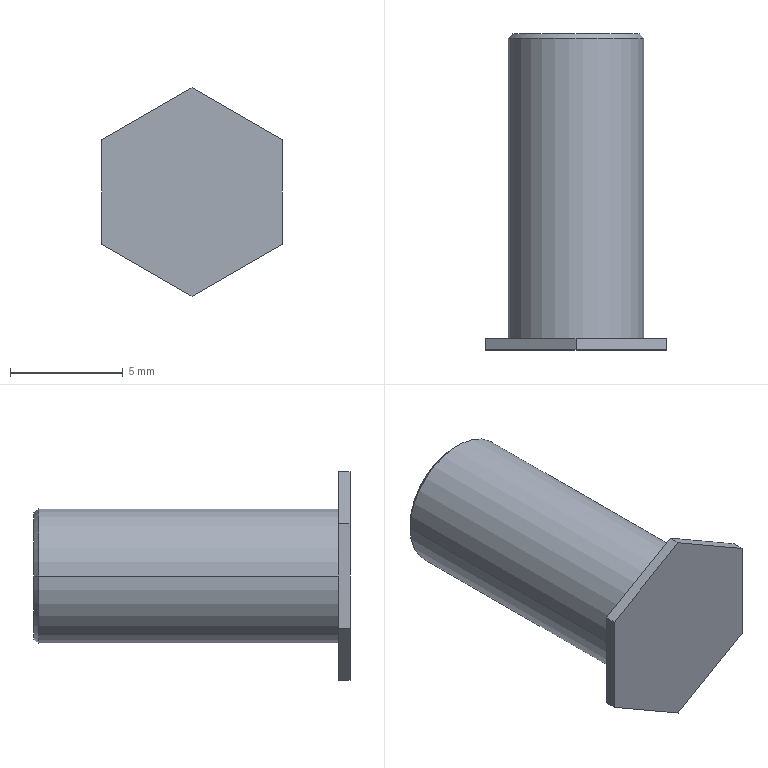Component | SolidWorks | FrontDoorAssembly-1_FrontDoorWelding-1_FrontDoorFrame(Riveted)PG50-02-101-1_FH-M6-14-1 | 1 solid | 13 faces | box 8 x 14 x 9.24 mm | volume 409 mm3 | plane 9 | cone 2 | cylinder 2 | commonest cylinder face diameters 6 x2
build123d program:
from build123d import *

# Parameters (mm, degrees)
BOSS_EXTRUDE1_DEPTH = 0.5
SKETCH2_R           = 3
BOSS_EXTRUDE2_DEPTH = 13.5
CHAMFER1_SIZE       = 0.2


with BuildPart() as part:
    # Sketch1 → Boss-Extrude1 (new body)
    with BuildSketch(Plane.XY):
        Polygon((0, 4.619), (-4, 2.309), (-4, -2.309), (0, -4.619), (4, -2.309), (4, 2.309), align=None)
    extrude(amount=BOSS_EXTRUDE1_DEPTH)

    # Sketch2 → Boss-Extrude2 (add)
    with BuildSketch(Plane.XY.offset(0.5)):
        Circle(SKETCH2_R)
    extrude(amount=BOSS_EXTRUDE2_DEPTH)

    # Chamfer1
    chamfer1_edges = [part.edges().sort_by_distance(p)[0] for p in [
        (-3, 0, 14),
    ]]
    chamfer(chamfer1_edges, length=CHAMFER1_SIZE)


solid = part.part

# Placed as in the assembly
solid = solid.moved(Location((897.314, -283.799, -334.996), (-90, 0, 0)))
STEP:
#1=CARTESIAN_POINT('',(35.438,-10.622,-13.189));
#2=VERTEX_POINT('',#1);
#3=CARTESIAN_POINT('',(35.217,-10.622,-13.189));
#4=VERTEX_POINT('',#3);
#5=CARTESIAN_POINT('',(35.327,-10.622,-13.189));
#6=DIRECTION('',(-0.,1.,0.));
#7=DIRECTION('',(1.,0.,0.));
#8=AXIS2_PLACEMENT_3D('',#5,#6,#7);
#9=CIRCLE('',#8,0.1102);
#10=EDGE_CURVE('',#2,#4,#9,.T.);
#11=ORIENTED_EDGE('',*,*,#10,.F.);
#12=CARTESIAN_POINT('',(35.445,-10.63,-13.189));
#13=VERTEX_POINT('',#12);
#14=CARTESIAN_POINT('',(35.438,-10.622,-13.189));
#15=DIRECTION('',(0.7071,-0.7071,-0.));
#16=VECTOR('',#15,39.37);
#17=LINE('',#14,#16);
#18=EDGE_CURVE('',#2,#13,#17,.T.);
#19=ORIENTED_EDGE('',*,*,#18,.T.);
#20=CARTESIAN_POINT('',(35.209,-10.63,-13.189));
#21=VERTEX_POINT('',#20);
#22=CARTESIAN_POINT('',(35.327,-10.63,-13.189));
#23=DIRECTION('',(0.,-1.,-0.));
#24=DIRECTION('',(1.,0.,0.));
#25=AXIS2_PLACEMENT_3D('',#22,#23,#24);
#26=CIRCLE('',#25,0.1181);
#27=EDGE_CURVE('',#21,#13,#26,.T.);
#28=ORIENTED_EDGE('',*,*,#27,.F.);
#29=CARTESIAN_POINT('',(35.217,-10.622,-13.189));
#30=DIRECTION('',(-0.7071,-0.7071,0.));
#31=VECTOR('',#30,39.37);
#32=LINE('',#29,#31);
#33=EDGE_CURVE('',#4,#21,#32,.T.);
#34=ORIENTED_EDGE('',*,*,#33,.F.);
#35=EDGE_LOOP('',(#11,#19,#28,#34));
#36=FACE_OUTER_BOUND('',#35,.T.);
#37=CARTESIAN_POINT('',(35.327,-10.622,-13.189));
#38=DIRECTION('',(0.,-1.,-0.));
#39=DIRECTION('',(-1.,0.,0.));
#40=AXIS2_PLACEMENT_3D('',#37,#38,#39);
#41=CONICAL_SURFACE('',#40,0.1102,0.7854);
#42=ADVANCED_FACE('',(#36),#41,.T.);
#43=ORIENTED_EDGE('',*,*,#27,.T.);
#44=CARTESIAN_POINT('',(35.445,-11.153,-13.189));
#45=VERTEX_POINT('',#44);
#46=CARTESIAN_POINT('',(35.445,-10.622,-13.189));
#47=DIRECTION('',(0.,-1.,-0.));
#48=VECTOR('',#47,39.37);
#49=LINE('',#46,#48);
#50=EDGE_CURVE('',#13,#45,#49,.T.);
#51=ORIENTED_EDGE('',*,*,#50,.T.);
#52=CARTESIAN_POINT('',(35.209,-11.153,-13.189));
#53=VERTEX_POINT('',#52);
#54=CARTESIAN_POINT('',(35.327,-11.153,-13.189));
#55=DIRECTION('',(-0.,1.,0.));
#56=DIRECTION('',(1.,0.,0.));
#57=AXIS2_PLACEMENT_3D('',#54,#55,#56);
#58=CIRCLE('',#57,0.1181);
#59=EDGE_CURVE('',#45,#53,#58,.T.);
#60=ORIENTED_EDGE('',*,*,#59,.T.);
#61=CARTESIAN_POINT('',(35.209,-10.622,-13.189));
#62=DIRECTION('',(0.,-1.,-0.));
#63=VECTOR('',#62,39.37);
#64=LINE('',#61,#63);
#65=EDGE_CURVE('',#21,#53,#64,.T.);
#66=ORIENTED_EDGE('',*,*,#65,.F.);
#67=EDGE_LOOP('',(#43,#51,#60,#66));
#68=FACE_OUTER_BOUND('',#67,.T.);
#69=CARTESIAN_POINT('',(35.327,-10.622,-13.189));
#70=DIRECTION('',(0.,-1.,-0.));
#71=DIRECTION('',(-1.,0.,0.));
#72=AXIS2_PLACEMENT_3D('',#69,#70,#71);
#73=CYLINDRICAL_SURFACE('',#72,0.1181);
#74=ADVANCED_FACE('',(#68),#73,.T.);
#75=CARTESIAN_POINT('',(35.485,-11.153,-13.28));
#76=VERTEX_POINT('',#75);
#77=CARTESIAN_POINT('',(35.327,-11.153,-13.371));
#78=VERTEX_POINT('',#77);
#79=CARTESIAN_POINT('',(35.485,-11.153,-13.28));
#80=DIRECTION('',(-0.866,-0.,-0.5));
#81=VECTOR('',#80,39.37);
#82=LINE('',#79,#81);
#83=EDGE_CURVE('',#76,#78,#82,.T.);
#84=ORIENTED_EDGE('',*,*,#83,.T.);
#85=CARTESIAN_POINT('',(35.17,-11.153,-13.28));
#86=VERTEX_POINT('',#85);
#87=CARTESIAN_POINT('',(35.327,-11.153,-13.371));
#88=DIRECTION('',(-0.866,-0.,0.5));
#89=VECTOR('',#88,39.37);
#90=LINE('',#87,#89);
#91=EDGE_CURVE('',#78,#86,#90,.T.);
#92=ORIENTED_EDGE('',*,*,#91,.T.);
#93=CARTESIAN_POINT('',(35.17,-11.153,-13.098));
#94=VERTEX_POINT('',#93);
#95=CARTESIAN_POINT('',(35.17,-11.153,-13.28));
#96=DIRECTION('',(-0.,-0.,1.));
#97=VECTOR('',#96,39.37);
#98=LINE('',#95,#97);
#99=EDGE_CURVE('',#86,#94,#98,.T.);
#100=ORIENTED_EDGE('',*,*,#99,.T.);
#101=CARTESIAN_POINT('',(35.327,-11.153,-13.007));
#102=VERTEX_POINT('',#101);
#103=CARTESIAN_POINT('',(35.17,-11.153,-13.098));
#104=DIRECTION('',(0.866,0.,0.5));
#105=VECTOR('',#104,39.37);
#106=LINE('',#103,#105);
#107=EDGE_CURVE('',#94,#102,#106,.T.);
#108=ORIENTED_EDGE('',*,*,#107,.T.);
#109=CARTESIAN_POINT('',(35.485,-11.153,-13.098));
#110=VERTEX_POINT('',#109);
#111=CARTESIAN_POINT('',(35.327,-11.153,-13.007));
#112=DIRECTION('',(0.866,0.,-0.5));
#113=VECTOR('',#112,39.37);
#114=LINE('',#111,#113);
#115=EDGE_CURVE('',#102,#110,#114,.T.);
#116=ORIENTED_EDGE('',*,*,#115,.T.);
#117=CARTESIAN_POINT('',(35.485,-11.153,-13.098));
#118=DIRECTION('',(-0.,-0.,-1.));
#119=VECTOR('',#118,39.37);
#120=LINE('',#117,#119);
#121=EDGE_CURVE('',#110,#76,#120,.T.);
#122=ORIENTED_EDGE('',*,*,#121,.T.);
#123=EDGE_LOOP('',(#84,#92,#100,#108,#116,#122));
#124=FACE_OUTER_BOUND('',#123,.T.);
#125=CARTESIAN_POINT('',(35.327,-11.153,-13.189));
#126=DIRECTION('',(-0.,1.,0.));
#127=DIRECTION('',(1.,0.,0.));
#128=AXIS2_PLACEMENT_3D('',#125,#126,#127);
#129=CIRCLE('',#128,0.1181);
#130=EDGE_CURVE('',#53,#45,#129,.T.);
#131=ORIENTED_EDGE('',*,*,#130,.F.);
#132=ORIENTED_EDGE('',*,*,#59,.F.);
#133=EDGE_LOOP('',(#131,#132));
#134=FACE_BOUND('',#133,.T.);
#135=CARTESIAN_POINT('',(35.327,-11.153,-13.371));
#136=DIRECTION('',(-0.,1.,0.));
#137=DIRECTION('',(1.,0.,-0.));
#138=AXIS2_PLACEMENT_3D('',#135,#136,#137);
#139=PLANE('',#138);
#140=ADVANCED_FACE('',(#124,#134),#139,.T.);
#141=CARTESIAN_POINT('',(35.485,-11.173,-13.28));
#142=VERTEX_POINT('',#141);
#143=CARTESIAN_POINT('',(35.327,-11.173,-13.371));
#144=VERTEX_POINT('',#143);
#145=CARTESIAN_POINT('',(35.485,-11.173,-13.28));
#146=DIRECTION('',(-0.866,-0.,-0.5));
#147=VECTOR('',#146,39.37);
#148=LINE('',#145,#147);
#149=EDGE_CURVE('',#142,#144,#148,.T.);
#150=ORIENTED_EDGE('',*,*,#149,.T.);
#151=CARTESIAN_POINT('',(35.327,-11.153,-13.371));
#152=DIRECTION('',(0.,-1.,-0.));
#153=VECTOR('',#152,39.37);
#154=LINE('',#151,#153);
#155=EDGE_CURVE('',#78,#144,#154,.T.);
#156=ORIENTED_EDGE('',*,*,#155,.F.);
#157=ORIENTED_EDGE('',*,*,#83,.F.);
#158=CARTESIAN_POINT('',(35.485,-11.153,-13.28));
#159=DIRECTION('',(0.,-1.,-0.));
#160=VECTOR('',#159,39.37);
#161=LINE('',#158,#160);
#162=EDGE_CURVE('',#76,#142,#161,.T.);
#163=ORIENTED_EDGE('',*,*,#162,.T.);
#164=EDGE_LOOP('',(#150,#156,#157,#163));
#165=FACE_OUTER_BOUND('',#164,.T.);
#166=CARTESIAN_POINT('',(35.485,-11.153,-13.28));
#167=DIRECTION('',(-0.5,-0.,0.866));
#168=DIRECTION('',(0.866,0.,0.5));
#169=AXIS2_PLACEMENT_3D('',#166,#167,#168);
#170=PLANE('',#169);
#171=ADVANCED_FACE('',(#165),#170,.F.);
#172=CARTESIAN_POINT('',(35.17,-11.173,-13.28));
#173=VERTEX_POINT('',#172);
#174=CARTESIAN_POINT('',(35.327,-11.173,-13.371));
#175=DIRECTION('',(-0.866,-0.,0.5));
#176=VECTOR('',#175,39.37);
#177=LINE('',#174,#176);
#178=EDGE_CURVE('',#144,#173,#177,.T.);
#179=ORIENTED_EDGE('',*,*,#178,.T.);
#180=CARTESIAN_POINT('',(35.17,-11.153,-13.28));
#181=DIRECTION('',(0.,-1.,-0.));
#182=VECTOR('',#181,39.37);
#183=LINE('',#180,#182);
#184=EDGE_CURVE('',#86,#173,#183,.T.);
#185=ORIENTED_EDGE('',*,*,#184,.F.);
#186=ORIENTED_EDGE('',*,*,#91,.F.);
#187=ORIENTED_EDGE('',*,*,#155,.T.);
#188=EDGE_LOOP('',(#179,#185,#186,#187));
#189=FACE_OUTER_BOUND('',#188,.T.);
#190=CARTESIAN_POINT('',(35.327,-11.153,-13.371));
#191=DIRECTION('',(0.5,0.,0.866));
#192=DIRECTION('',(0.866,0.,-0.5));
#193=AXIS2_PLACEMENT_3D('',#190,#191,#192);
#194=PLANE('',#193);
#195=ADVANCED_FACE('',(#189),#194,.F.);
#196=CARTESIAN_POINT('',(35.17,-11.173,-13.098));
#197=VERTEX_POINT('',#196);
#198=CARTESIAN_POINT('',(35.17,-11.173,-13.28));
#199=DIRECTION('',(-0.,-0.,1.));
#200=VECTOR('',#199,39.37);
#201=LINE('',#198,#200);
#202=EDGE_CURVE('',#173,#197,#201,.T.);
#203=ORIENTED_EDGE('',*,*,#202,.T.);
#204=CARTESIAN_POINT('',(35.17,-11.153,-13.098));
#205=DIRECTION('',(0.,-1.,-0.));
#206=VECTOR('',#205,39.37);
#207=LINE('',#204,#206);
#208=EDGE_CURVE('',#94,#197,#207,.T.);
#209=ORIENTED_EDGE('',*,*,#208,.F.);
#210=ORIENTED_EDGE('',*,*,#99,.F.);
#211=ORIENTED_EDGE('',*,*,#184,.T.);
#212=EDGE_LOOP('',(#203,#209,#210,#211));
#213=FACE_OUTER_BOUND('',#212,.T.);
#214=CARTESIAN_POINT('',(35.17,-11.153,-13.28));
#215=DIRECTION('',(1.,0.,0.));
#216=DIRECTION('',(0.,0.,-1.));
#217=AXIS2_PLACEMENT_3D('',#214,#215,#216);
#218=PLANE('',#217);
#219=ADVANCED_FACE('',(#213),#218,.F.);
#220=CARTESIAN_POINT('',(35.327,-11.173,-13.007));
#221=VERTEX_POINT('',#220);
#222=CARTESIAN_POINT('',(35.17,-11.173,-13.098));
#223=DIRECTION('',(0.866,0.,0.5));
#224=VECTOR('',#223,39.37);
#225=LINE('',#222,#224);
#226=EDGE_CURVE('',#197,#221,#225,.T.);
#227=ORIENTED_EDGE('',*,*,#226,.T.);
#228=CARTESIAN_POINT('',(35.327,-11.153,-13.007));
#229=DIRECTION('',(0.,-1.,-0.));
#230=VECTOR('',#229,39.37);
#231=LINE('',#228,#230);
#232=EDGE_CURVE('',#102,#221,#231,.T.);
#233=ORIENTED_EDGE('',*,*,#232,.F.);
#234=ORIENTED_EDGE('',*,*,#107,.F.);
#235=ORIENTED_EDGE('',*,*,#208,.T.);
#236=EDGE_LOOP('',(#227,#233,#234,#235));
#237=FACE_OUTER_BOUND('',#236,.T.);
#238=CARTESIAN_POINT('',(35.17,-11.153,-13.098));
#239=DIRECTION('',(0.5,0.,-0.866));
#240=DIRECTION('',(-0.866,-0.,-0.5));
#241=AXIS2_PLACEMENT_3D('',#238,#239,#240);
#242=PLANE('',#241);
#243=ADVANCED_FACE('',(#237),#242,.F.);
#244=CARTESIAN_POINT('',(35.485,-11.173,-13.098));
#245=VERTEX_POINT('',#244);
#246=CARTESIAN_POINT('',(35.327,-11.173,-13.007));
#247=DIRECTION('',(0.866,0.,-0.5));
#248=VECTOR('',#247,39.37);
#249=LINE('',#246,#248);
#250=EDGE_CURVE('',#221,#245,#249,.T.);
#251=ORIENTED_EDGE('',*,*,#250,.T.);
#252=CARTESIAN_POINT('',(35.485,-11.153,-13.098));
#253=DIRECTION('',(0.,-1.,-0.));
#254=VECTOR('',#253,39.37);
#255=LINE('',#252,#254);
#256=EDGE_CURVE('',#110,#245,#255,.T.);
#257=ORIENTED_EDGE('',*,*,#256,.F.);
#258=ORIENTED_EDGE('',*,*,#115,.F.);
#259=ORIENTED_EDGE('',*,*,#232,.T.);
#260=EDGE_LOOP('',(#251,#257,#258,#259));
#261=FACE_OUTER_BOUND('',#260,.T.);
#262=CARTESIAN_POINT('',(35.327,-11.153,-13.007));
#263=DIRECTION('',(-0.5,-0.,-0.866));
#264=DIRECTION('',(-0.866,-0.,0.5));
#265=AXIS2_PLACEMENT_3D('',#262,#263,#264);
#266=PLANE('',#265);
#267=ADVANCED_FACE('',(#261),#266,.F.);
#268=CARTESIAN_POINT('',(35.485,-11.173,-13.098));
#269=DIRECTION('',(-0.,-0.,-1.));
#270=VECTOR('',#269,39.37);
#271=LINE('',#268,#270);
#272=EDGE_CURVE('',#245,#142,#271,.T.);
#273=ORIENTED_EDGE('',*,*,#272,.T.);
#274=ORIENTED_EDGE('',*,*,#162,.F.);
#275=ORIENTED_EDGE('',*,*,#121,.F.);
#276=ORIENTED_EDGE('',*,*,#256,.T.);
#277=EDGE_LOOP('',(#273,#274,#275,#276));
#278=FACE_OUTER_BOUND('',#277,.T.);
#279=CARTESIAN_POINT('',(35.485,-11.153,-13.098));
#280=DIRECTION('',(-1.,-0.,0.));
#281=DIRECTION('',(0.,0.,1.));
#282=AXIS2_PLACEMENT_3D('',#279,#280,#281);
#283=PLANE('',#282);
#284=ADVANCED_FACE('',(#278),#283,.F.);
#285=ORIENTED_EDGE('',*,*,#149,.F.);
#286=ORIENTED_EDGE('',*,*,#272,.F.);
#287=ORIENTED_EDGE('',*,*,#250,.F.);
#288=ORIENTED_EDGE('',*,*,#226,.F.);
#289=ORIENTED_EDGE('',*,*,#202,.F.);
#290=ORIENTED_EDGE('',*,*,#178,.F.);
#291=EDGE_LOOP('',(#285,#286,#287,#288,#289,#290));
#292=FACE_OUTER_BOUND('',#291,.T.);
#293=CARTESIAN_POINT('',(35.327,-11.173,-13.371));
#294=DIRECTION('',(-0.,1.,0.));
#295=DIRECTION('',(1.,0.,-0.));
#296=AXIS2_PLACEMENT_3D('',#293,#294,#295);
#297=PLANE('',#296);
#298=ADVANCED_FACE('',(#292),#297,.F.);
#299=ORIENTED_EDGE('',*,*,#50,.F.);
#300=CARTESIAN_POINT('',(35.327,-10.63,-13.189));
#301=DIRECTION('',(0.,-1.,-0.));
#302=DIRECTION('',(1.,0.,0.));
#303=AXIS2_PLACEMENT_3D('',#300,#301,#302);
#304=CIRCLE('',#303,0.1181);
#305=EDGE_CURVE('',#13,#21,#304,.T.);
#306=ORIENTED_EDGE('',*,*,#305,.T.);
#307=ORIENTED_EDGE('',*,*,#65,.T.);
#308=ORIENTED_EDGE('',*,*,#130,.T.);
#309=EDGE_LOOP('',(#299,#306,#307,#308));
#310=FACE_OUTER_BOUND('',#309,.T.);
#311=CARTESIAN_POINT('',(35.327,-10.622,-13.189));
#312=DIRECTION('',(0.,-1.,-0.));
#313=DIRECTION('',(-1.,0.,0.));
#314=AXIS2_PLACEMENT_3D('',#311,#312,#313);
#315=CYLINDRICAL_SURFACE('',#314,0.1181);
#316=ADVANCED_FACE('',(#310),#315,.T.);
#317=CARTESIAN_POINT('',(35.327,-10.622,-13.189));
#318=DIRECTION('',(-0.,1.,0.));
#319=DIRECTION('',(1.,0.,0.));
#320=AXIS2_PLACEMENT_3D('',#317,#318,#319);
#321=CIRCLE('',#320,0.1102);
#322=EDGE_CURVE('',#4,#2,#321,.T.);
#323=ORIENTED_EDGE('',*,*,#322,.T.);
#324=ORIENTED_EDGE('',*,*,#10,.T.);
#325=EDGE_LOOP('',(#323,#324));
#326=FACE_OUTER_BOUND('',#325,.T.);
#327=CARTESIAN_POINT('',(35.327,-10.622,-13.189));
#328=DIRECTION('',(-0.,1.,0.));
#329=DIRECTION('',(1.,0.,-0.));
#330=AXIS2_PLACEMENT_3D('',#327,#328,#329);
#331=PLANE('',#330);
#332=ADVANCED_FACE('',(#326),#331,.T.);
#333=ORIENTED_EDGE('',*,*,#18,.F.);
#334=ORIENTED_EDGE('',*,*,#322,.F.);
#335=ORIENTED_EDGE('',*,*,#33,.T.);
#336=ORIENTED_EDGE('',*,*,#305,.F.);
#337=EDGE_LOOP('',(#333,#334,#335,#336));
#338=FACE_OUTER_BOUND('',#337,.T.);
#339=CARTESIAN_POINT('',(35.327,-10.622,-13.189));
#340=DIRECTION('',(0.,-1.,-0.));
#341=DIRECTION('',(-1.,0.,0.));
#342=AXIS2_PLACEMENT_3D('',#339,#340,#341);
#343=CONICAL_SURFACE('',#342,0.1102,0.7854);
#344=ADVANCED_FACE('',(#338),#343,.T.);
#345=CLOSED_SHELL('',(#42,#74,#140,#171,#195,#219,#243,#267,#284,#298,#316,#332,#344));
#346=MANIFOLD_SOLID_BREP('',#345);
#347=CARTESIAN_POINT('',(0.,0.,0.));
#348=DIRECTION('',(0.,0.,1.));
#349=DIRECTION('',(1.,0.,0.));
#350=AXIS2_PLACEMENT_3D('',#347,#348,#349);
#351=(LENGTH_UNIT()NAMED_UNIT(*)SI_UNIT($,.METRE.));
#352=LENGTH_MEASURE_WITH_UNIT(LENGTH_MEASURE(0.0254),#351);
#353=DIMENSIONAL_EXPONENTS(1.,0.,0.,0.,0.,0.,0.);
#354=(CONVERSION_BASED_UNIT('',#352)LENGTH_UNIT()NAMED_UNIT(#353));
#355=UNCERTAINTY_MEASURE_WITH_UNIT(LENGTH_MEASURE(0.00001),#354,'','');
#356=(NAMED_UNIT(*)PLANE_ANGLE_UNIT()SI_UNIT($,.RADIAN.));
#357=(NAMED_UNIT(*)SI_UNIT($,.STERADIAN.)SOLID_ANGLE_UNIT());
#358=(GEOMETRIC_REPRESENTATION_CONTEXT(3)GLOBAL_UNCERTAINTY_ASSIGNED_CONTEXT((#355))GLOBAL_UNIT_ASSIGNED_CONTEXT((#354,#356,#357))REPRESENTATION_CONTEXT('',''));
#359=ADVANCED_BREP_SHAPE_REPRESENTATION('',(#346,#350),#358);
#360=COLOUR_RGB('',0.7922,0.8196,0.9333);
#361=FILL_AREA_STYLE_COLOUR('',#360);
#362=FILL_AREA_STYLE('',(#361));
#363=SURFACE_STYLE_FILL_AREA(#362);
#364=SURFACE_SIDE_STYLE('',(#363));
#365=SURFACE_STYLE_USAGE(.BOTH.,#364);
#366=PRESENTATION_STYLE_ASSIGNMENT((#365));
#367=STYLED_ITEM('',(#366),#346);
#368=PRESENTATION_LAYER_ASSIGNMENT('','',(#367));
#369=(LENGTH_UNIT()NAMED_UNIT(*)SI_UNIT($,.METRE.));
#370=LENGTH_MEASURE_WITH_UNIT(LENGTH_MEASURE(0.0254),#369);
#371=DIMENSIONAL_EXPONENTS(1.,0.,0.,0.,0.,0.,0.);
#372=(CONVERSION_BASED_UNIT('',#370)LENGTH_UNIT()NAMED_UNIT(#371));
#373=UNCERTAINTY_MEASURE_WITH_UNIT(LENGTH_MEASURE(0.00001),#372,'','');
#374=(NAMED_UNIT(*)PLANE_ANGLE_UNIT()SI_UNIT($,.RADIAN.));
#375=(NAMED_UNIT(*)SI_UNIT($,.STERADIAN.)SOLID_ANGLE_UNIT());
#376=(GEOMETRIC_REPRESENTATION_CONTEXT(3)GLOBAL_UNCERTAINTY_ASSIGNED_CONTEXT((#373))GLOBAL_UNIT_ASSIGNED_CONTEXT((#372,#374,#375))REPRESENTATION_CONTEXT('',''));
#377=MECHANICAL_DESIGN_GEOMETRIC_PRESENTATION_REPRESENTATION('',(#367),#376);